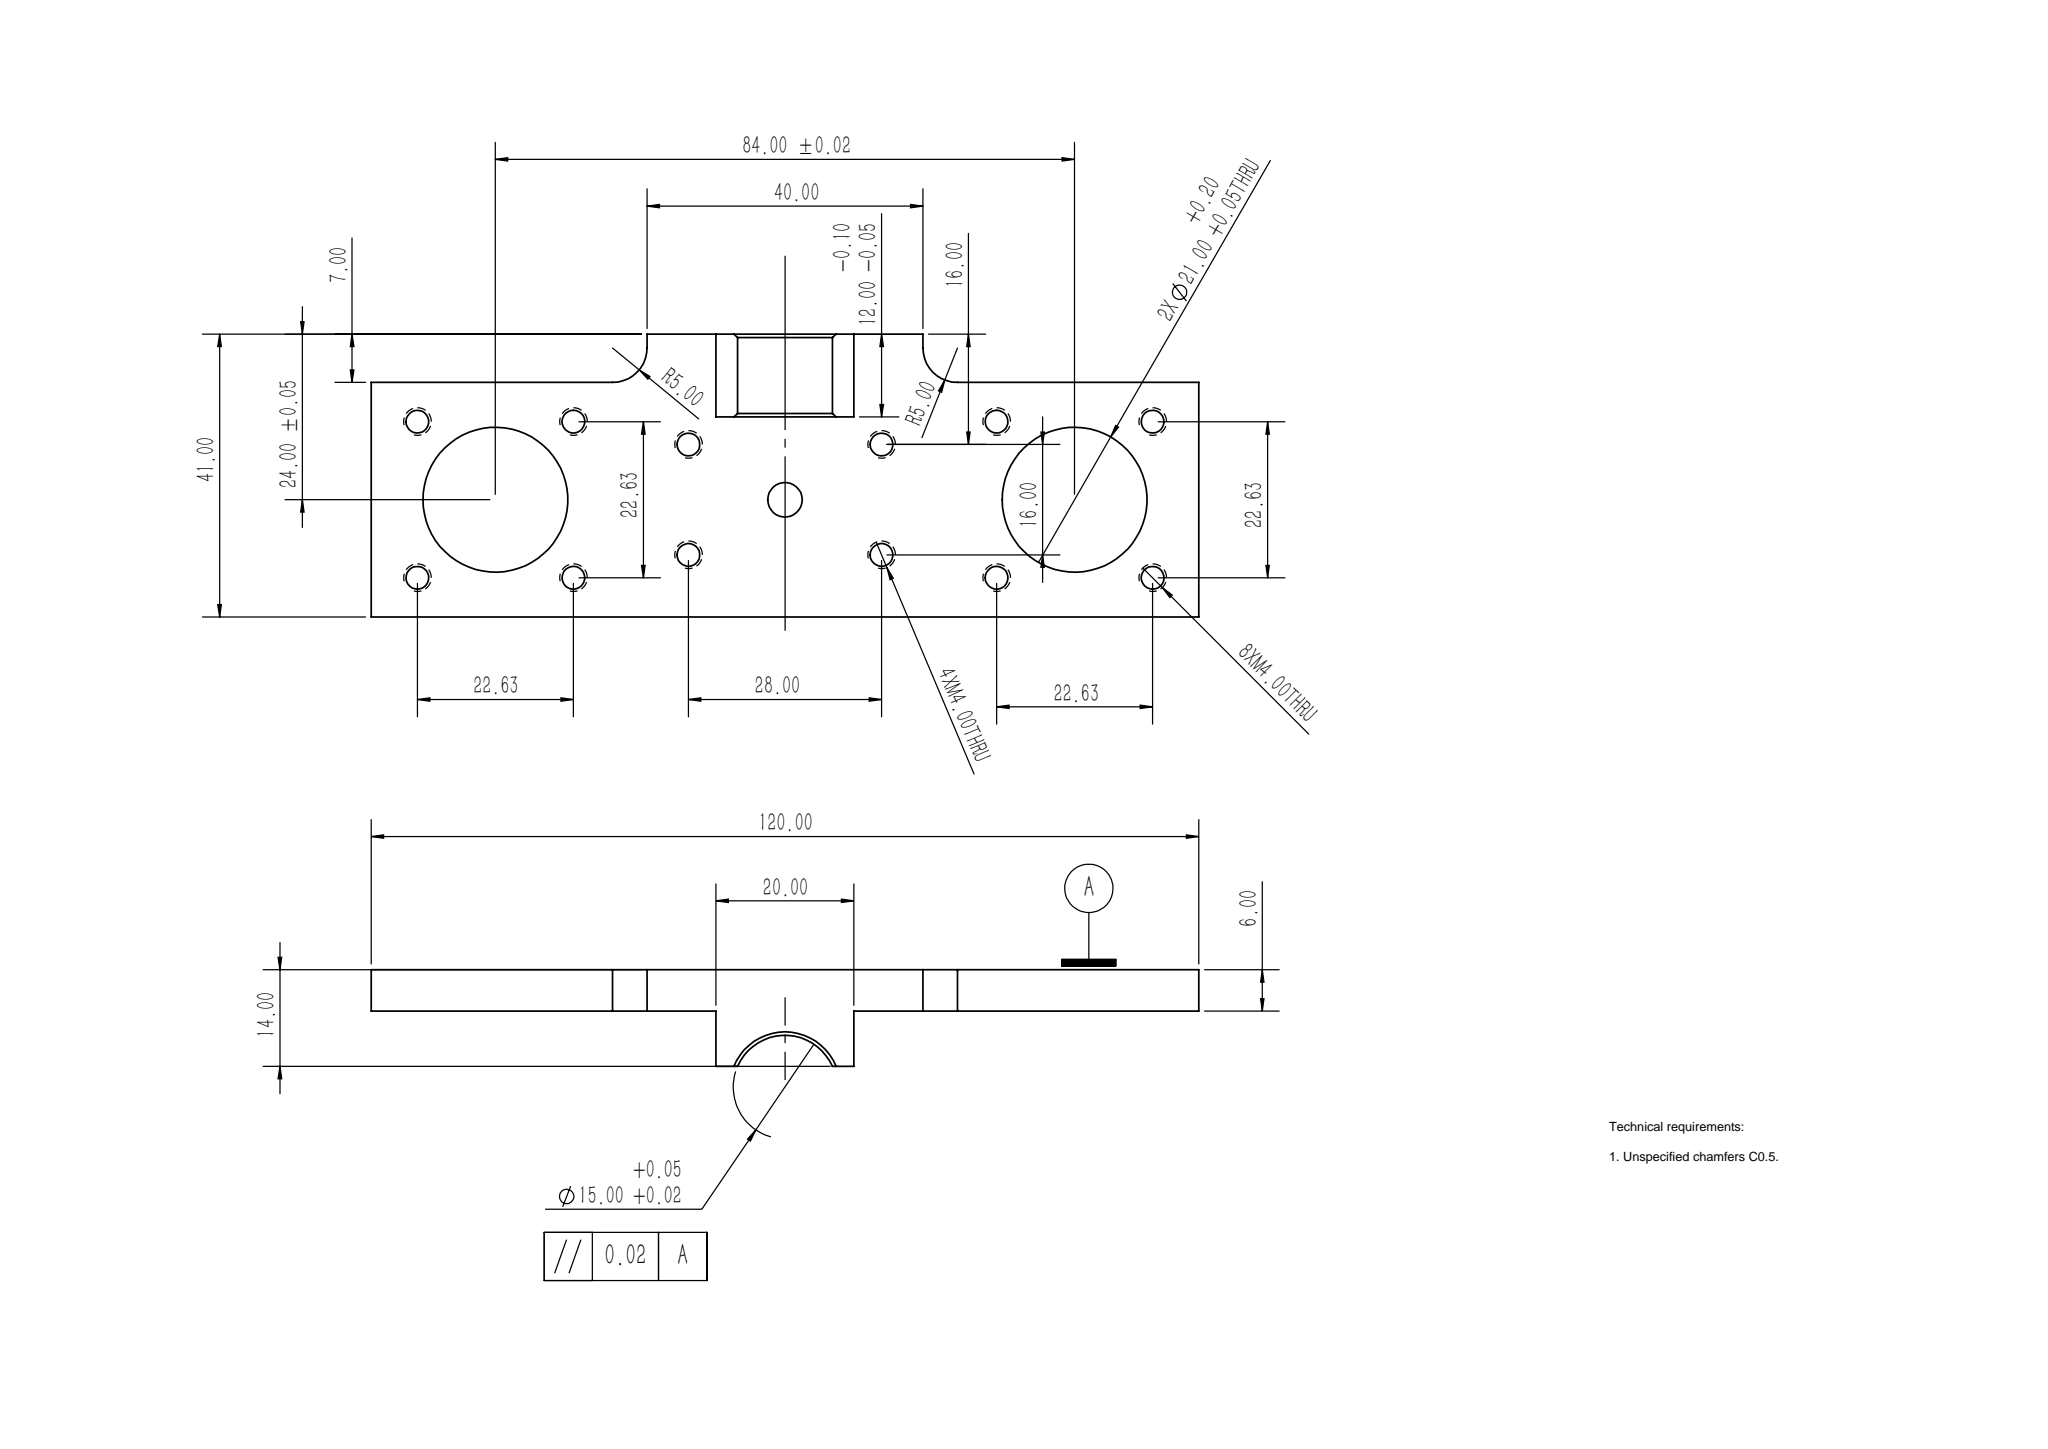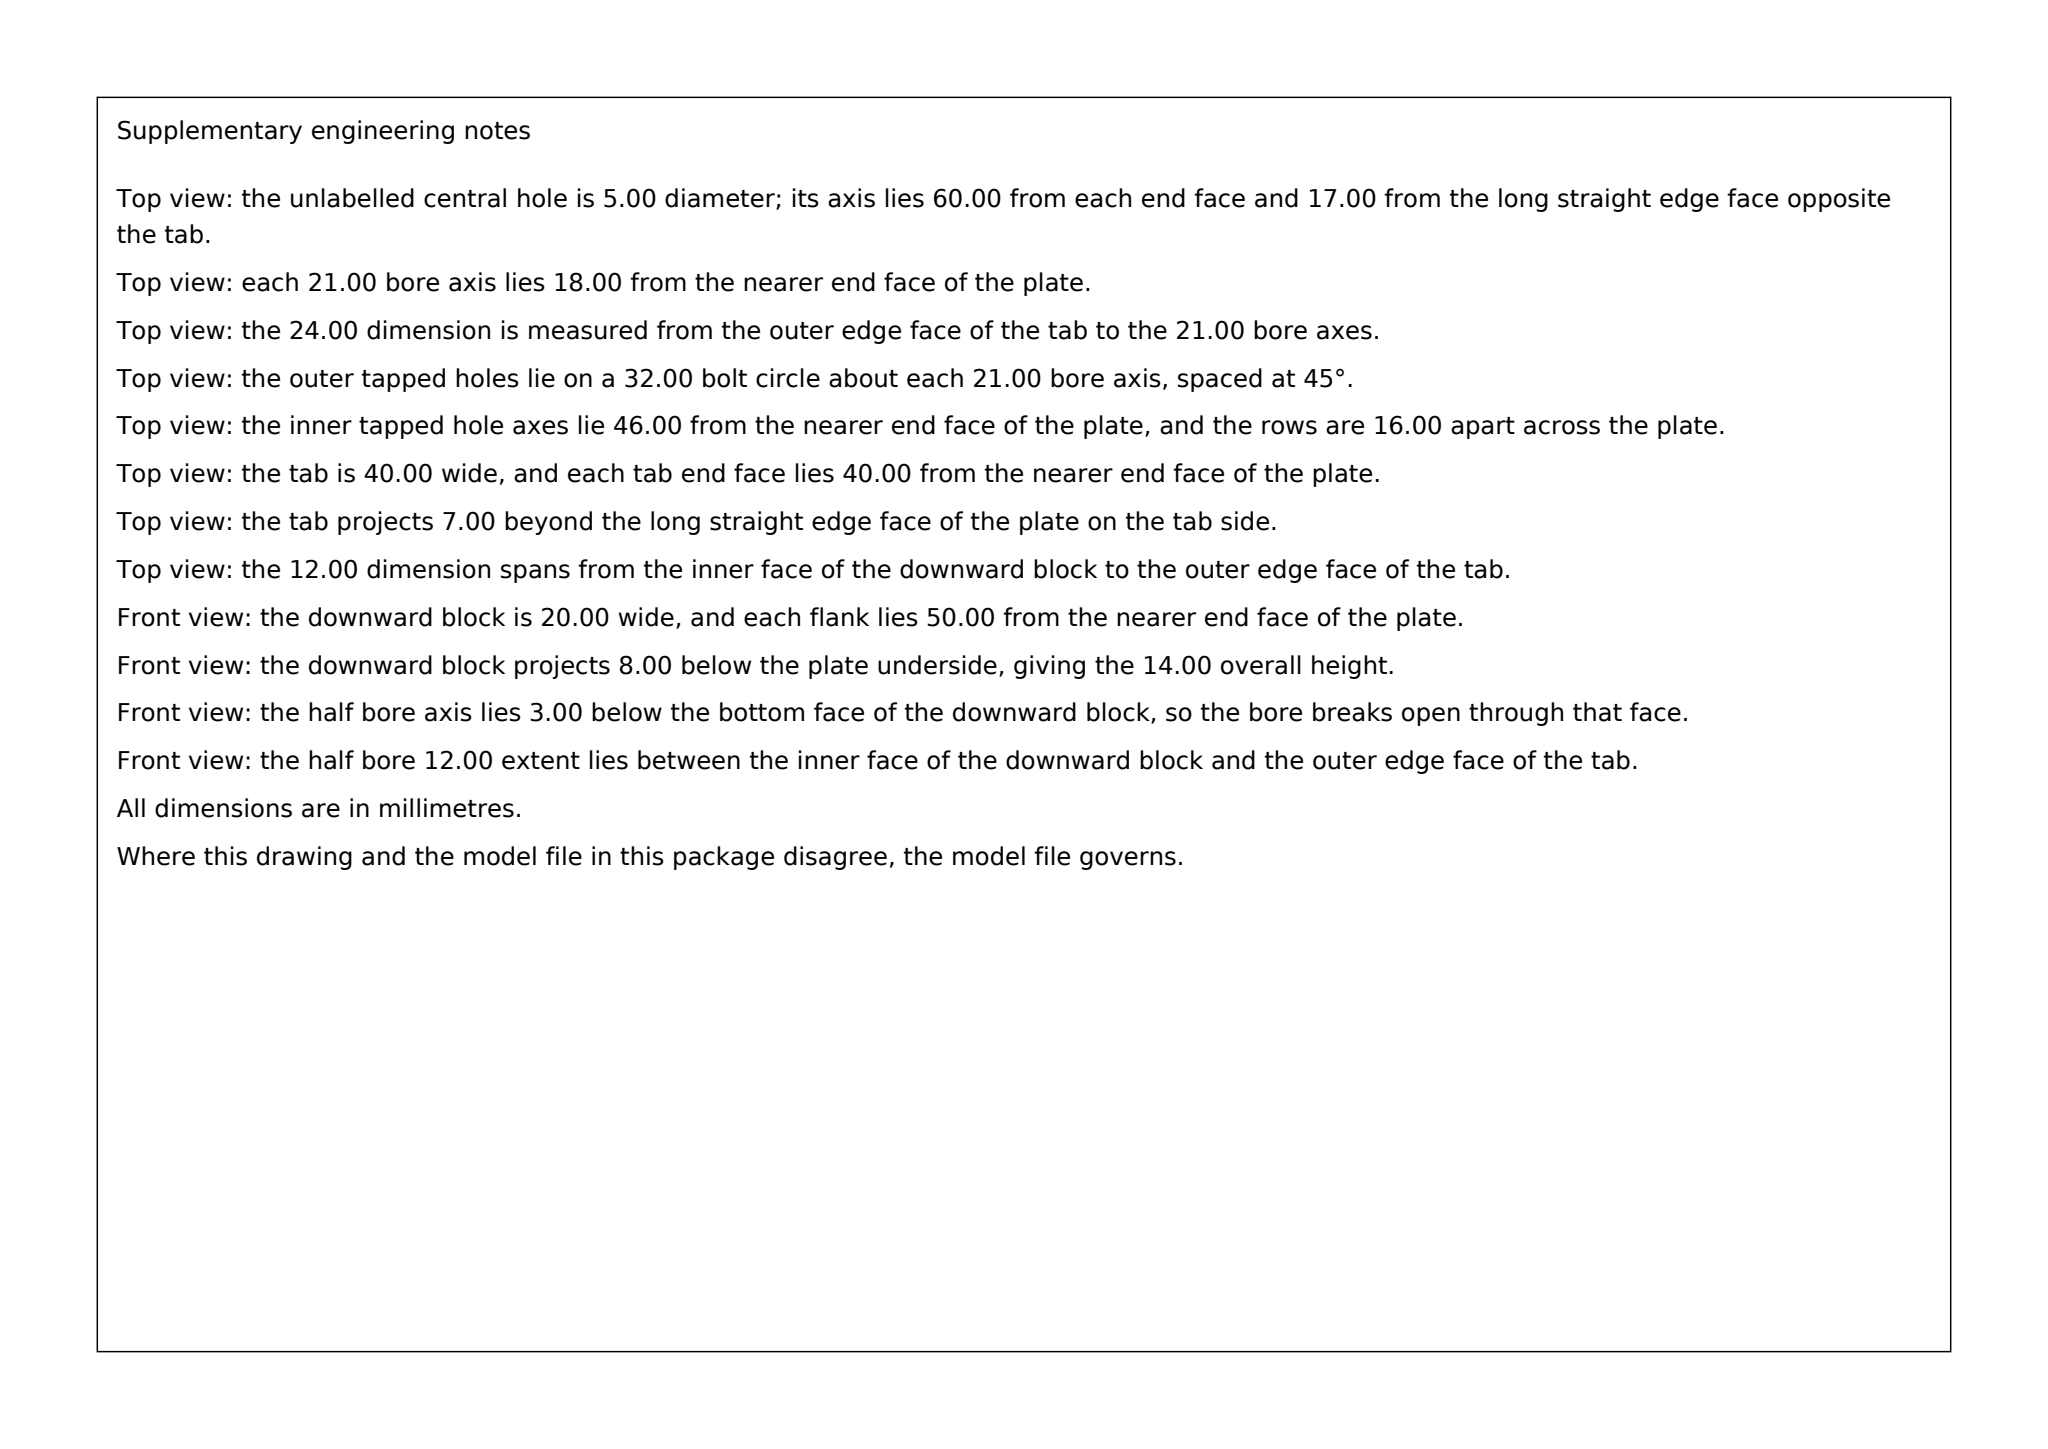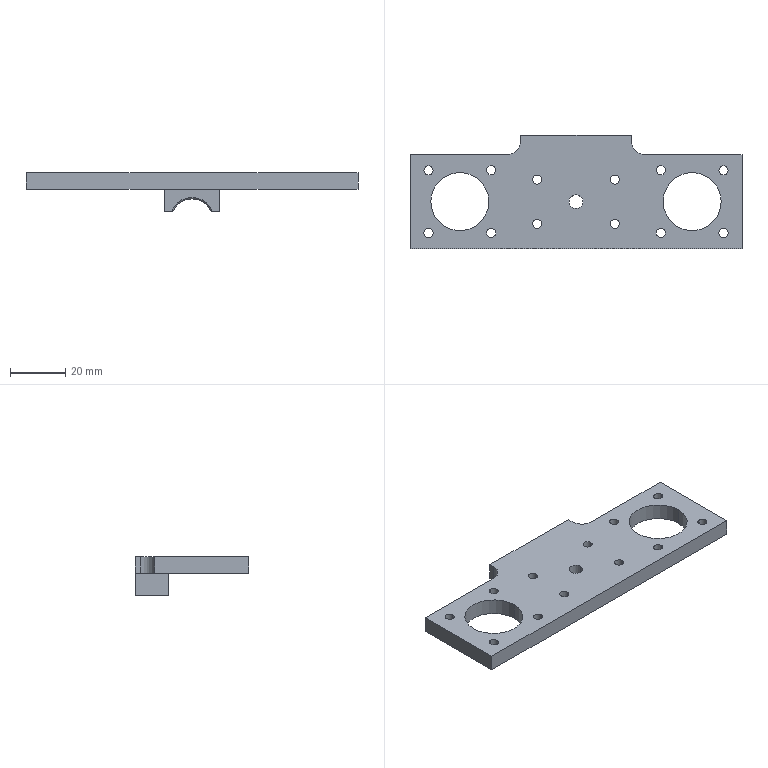Part | SolidWorks | mm | 1 solid | 50 faces | box 120 x 41 x 14 mm | volume 22715 mm3 | cylinder 33 | plane 15 | cone 2 | commonest cylinder face diameters 3.3 x24 21 x4 5 x2 10 x2 15 x1
Drawing notes:
Ø5.00 THRU C/L 24.00 FROM TOP EDGE, COMMON W/ Ø21 BORE C/L | from the solid: Ø5.0 z-cyl at (60,17); bbox Y=41 so 41-17=24 from top edge, same Y as Ø21 bores at y=17
8XM4.00 THRU: 22.63 x 22.63 SQ PATTERN CONC W/ Ø21 BORES | from the solid: Ø3.3 holes at (6.69/29.31, 5.69/28.31) ctr (18,17) and (90.69/113.31, 5.69/28.31) ctr (102,17) = Ø21 bore axes
4XM4.00 THRU, 28.00 x 16.00 CTRS, SYM ABOUT PART C/L | from the solid: Ø3.3 holes at (46,9),(46,25),(74,9),(74,25); spacing 28 in X, 16 in Y, centred on x=60, y=17
build123d program:
from build123d import *

# Parameters (mm, degrees)
SKETCH1_W             = 120
SKETCH1_H             = 48
BOSS_EXTRUDE1_DEPTH   = 14
SKETCH2_W             = 50
SKETCH2_H             = 8
CUT_EXTRUDE1_DEPTH    = 79.102
SKETCH5_R             = 7.5
CUT_EXTRUDE2_DEPTH    = 79.102
SKETCH6_W             = 20
SKETCH6_H             = 36
CUT_EXTRUDE3_DEPTH    = 8
M4_TAPPED_HOLE1_D     = 3.3
M4_TAPPED_HOLE1_DEPTH = 10.1
M4_TAPPED_HOLE1_TIP   = 0.9914
SKETCH9_R             = 10.5
CUT_EXTRUDE4_DEPTH    = 67.121
SKETCH10_R            = 2.5
CUT_EXTRUDE5_DEPTH    = 67.121
SKETCH11_W            = 120
SKETCH11_H            = 7
CUT_EXTRUDE6_DEPTH    = 67.121
SKETCH12_W            = 40
SKETCH12_H            = 7
CUT_EXTRUDE7_DEPTH    = 67.121
CIRPATTERN1_COUNT     = 4
FILLET1_R             = 5
CHAMFER1_SIZE         = 0.5


with BuildPart() as part:
    # Sketch1 → Boss-Extrude1 (new body)
    with BuildSketch(Plane.XY):
        Rectangle(SKETCH1_W, SKETCH1_H)
    extrude(amount=BOSS_EXTRUDE1_DEPTH)

    # Sketch2 → Cut-Extrude1 (cut, through all)
    with BuildSketch(Plane(origin=(0, 24, 0), x_dir=(1, 0, 0), z_dir=(0, 1, 0))):
        with Locations((-35, -4)):
            Rectangle(SKETCH2_W, SKETCH2_H)
        with Locations((35, -4)):
            Rectangle(SKETCH2_W, SKETCH2_H)
    extrude(amount=-CUT_EXTRUDE1_DEPTH, mode=Mode.SUBTRACT)

    # Sketch5 → Cut-Extrude2 (cut, through all)
    with BuildSketch(Plane(origin=(0, 24, 0), x_dir=(1, 0, 0), z_dir=(0, 1, 0))):
        with Locations((0, 3)):
            Circle(SKETCH5_R)
    extrude(amount=-CUT_EXTRUDE2_DEPTH, mode=Mode.SUBTRACT)

    # Sketch6 → Cut-Extrude3 (cut)
    with BuildSketch(Plane(origin=(0, 0, 0), x_dir=(-1, 0, 0), z_dir=(0, 0, -1))):
        with Locations((0, -6)):
            Rectangle(SKETCH6_W, SKETCH6_H)
    extrude(amount=-CUT_EXTRUDE3_DEPTH, mode=Mode.SUBTRACT)

    # M4 Tapped Hole1
    with Locations(Plane.XY.offset(14)):
        with Locations((14, 8), (14, -8), (-14, -8), (-14, 8)):
            Hole(M4_TAPPED_HOLE1_D / 2, depth=M4_TAPPED_HOLE1_DEPTH)
            with Locations((0, 0, -(M4_TAPPED_HOLE1_DEPTH + M4_TAPPED_HOLE1_TIP / 2))):  # 118° drill point
                Cone(0, M4_TAPPED_HOLE1_D / 2, M4_TAPPED_HOLE1_TIP, mode=Mode.SUBTRACT)

    # Sketch9 → Cut-Extrude4 (cut, through all)
    with BuildSketch(Plane.XY.offset(14)):
        with Locations((-42, 0)):
            Circle(SKETCH9_R)
        with Locations((42, 0)):
            Circle(SKETCH9_R)
    extrude(amount=-CUT_EXTRUDE4_DEPTH, mode=Mode.SUBTRACT)

    # Sketch10 → Cut-Extrude5 (cut, through all)
    with BuildSketch(Plane.XY.offset(14)):
        Circle(SKETCH10_R)
    extrude(amount=-CUT_EXTRUDE5_DEPTH, mode=Mode.SUBTRACT)

    # Sketch11 → Cut-Extrude6 (cut, through all)
    with BuildSketch(Plane.XY.offset(14)):
        with Locations((0, -20.5)):
            Rectangle(SKETCH11_W, SKETCH11_H)
    extrude(amount=-CUT_EXTRUDE6_DEPTH, mode=Mode.SUBTRACT)

    # Sketch12 → Cut-Extrude7 (cut, through all)
    with BuildSketch(Plane.XY.offset(14)):
        with Locations((-40, 20.5)):
            Rectangle(SKETCH12_W, SKETCH12_H)
        with Locations((40, 20.5)):
            Rectangle(SKETCH12_W, SKETCH12_H)
    extrude(amount=-CUT_EXTRUDE7_DEPTH, mode=Mode.SUBTRACT)

    # Sketch13 → M4 Tapped Hole2 (revolve, cut)
    with BuildSketch(Plane(origin=(53.314, 11.314, 14), x_dir=(0, -1, 0), z_dir=(1, 0, 0))):
        Polygon((0, 0), (0, 11.091), (1.65, 10.1), (1.65, 0), align=None)
    m4_tapped_hole2 = revolve(axis=Axis((53.314, 11.314, 20.35), (0, 0, -1)), mode=Mode.SUBTRACT)

    # CirPattern1: M4 Tapped Hole2 ×4 about axis
    cirpattern1_axis = Axis((42, 0, 0), (0, 0, 1))
    for i in range(1, CIRPATTERN1_COUNT):
        add(m4_tapped_hole2.rotate(cirpattern1_axis, i * 360 / CIRPATTERN1_COUNT), mode=Mode.SUBTRACT)

    # Mirror1: M4 Tapped Hole2 across plane
    add(m4_tapped_hole2.mirror(Plane(origin=(0, 0, 0), x_dir=(0, 0, 1), z_dir=(1, 0, 0))), mode=Mode.SUBTRACT)

    # Mirror1 copy 1 sketch → Mirror1 copy 1 (revolve, cut)
    with BuildSketch(Plane(origin=(-30.686, 11.314, 14), x_dir=(-1, 0, 0), z_dir=(0, 1, 0))):
        Polygon((0, 0), (0, -11.091), (1.65, -10.1), (1.65, 0), align=None)
    revolve(axis=Axis((-30.686, 11.314, 20.35), (0, 0, 1)), mode=Mode.SUBTRACT)

    # Mirror1 copy 2 sketch → Mirror1 copy 2 (revolve, cut)
    with BuildSketch(Plane(origin=(-30.686, -11.314, 14), x_dir=(0, 1, 0), z_dir=(1, 0, 0))):
        Polygon((0, 0), (0, -11.091), (1.65, -10.1), (1.65, 0), align=None)
    revolve(axis=Axis((-30.686, -11.314, 20.35), (0, 0, 1)), mode=Mode.SUBTRACT)

    # Mirror1 copy 3 sketch → Mirror1 copy 3 (revolve, cut)
    with BuildSketch(Plane(origin=(-53.314, -11.314, 14), x_dir=(1, 0, 0), z_dir=(0, -1, 0))):
        Polygon((0, 0), (0, -11.091), (1.65, -10.1), (1.65, 0), align=None)
    revolve(axis=Axis((-53.314, -11.314, 20.35), (0, 0, 1)), mode=Mode.SUBTRACT)

    # Fillet1
    fillet1_edges = [part.edges().sort_by_distance(p)[0] for p in [
        (-20, 17, 11),
        (20, 17, 11),
    ]]
    fillet(fillet1_edges, radius=FILLET1_R)

    # Chamfer1
    chamfer1_edges = [part.edges().sort_by_distance(p)[0] for p in [
        (0, 24, 4.5),
        (0, 12, 4.5),
    ]]
    chamfer(chamfer1_edges, length=CHAMFER1_SIZE)


solid = part.part